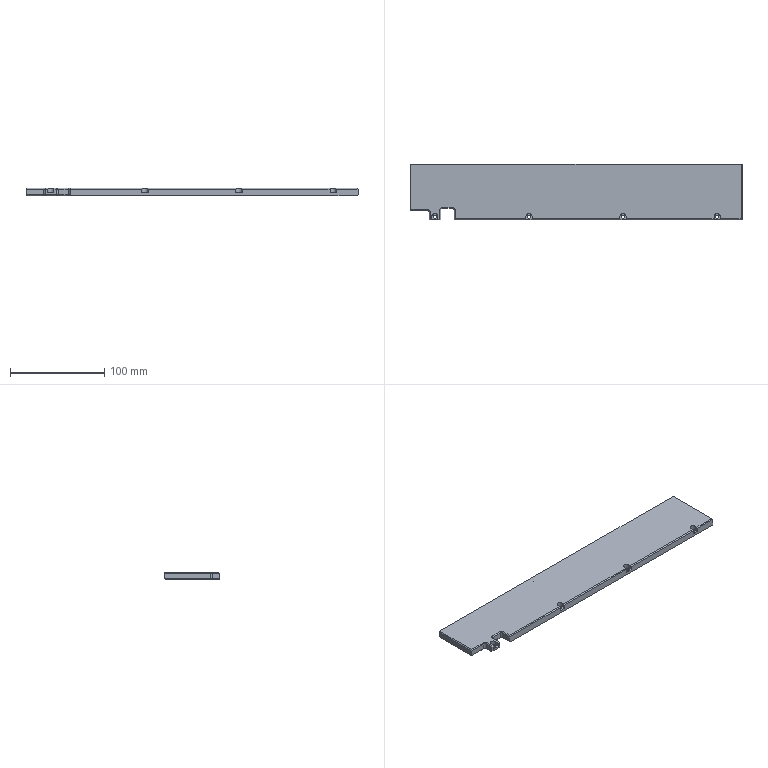CAM job | Mastercam | mm | 9 operations | part box 353 x 59 x 8
1. Contour (2D) | 7 - 4 平底刀
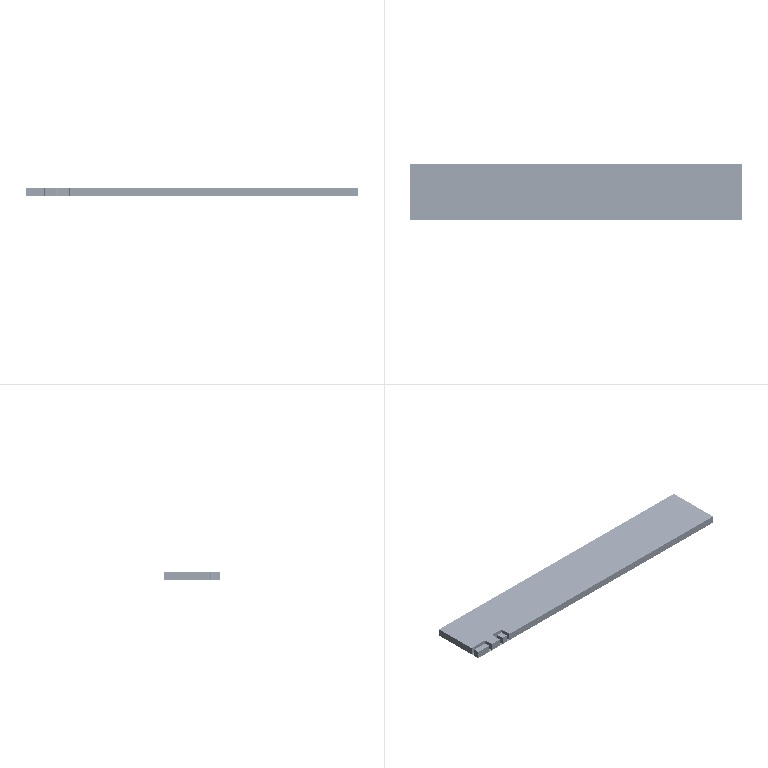2. Contour (Ramp) | 7 - 4 平底刀
3. Contour (2D) | 7 - 4 平底刀
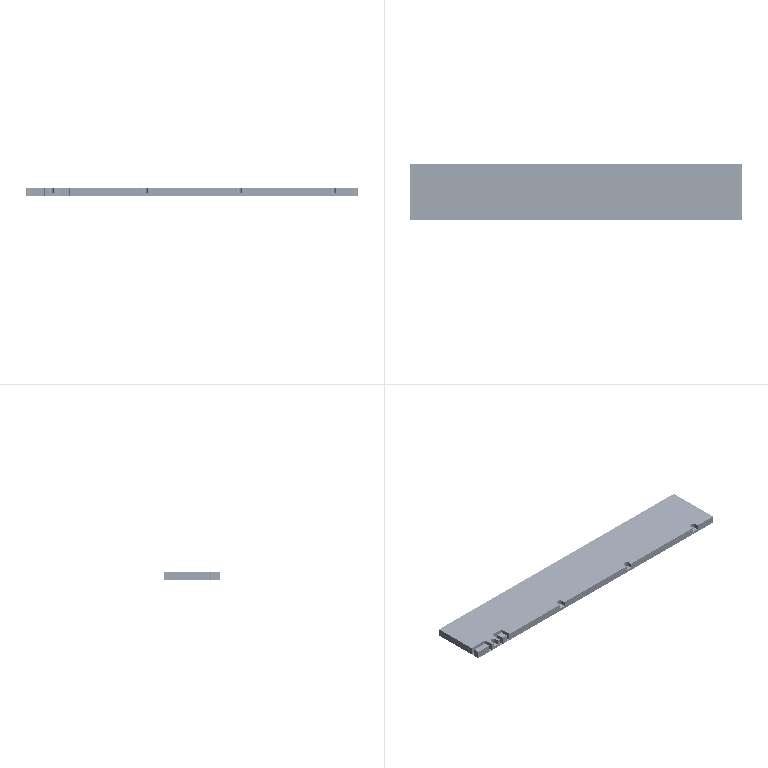4. Contour (2D chamfer) | 2 - 4定位倒角
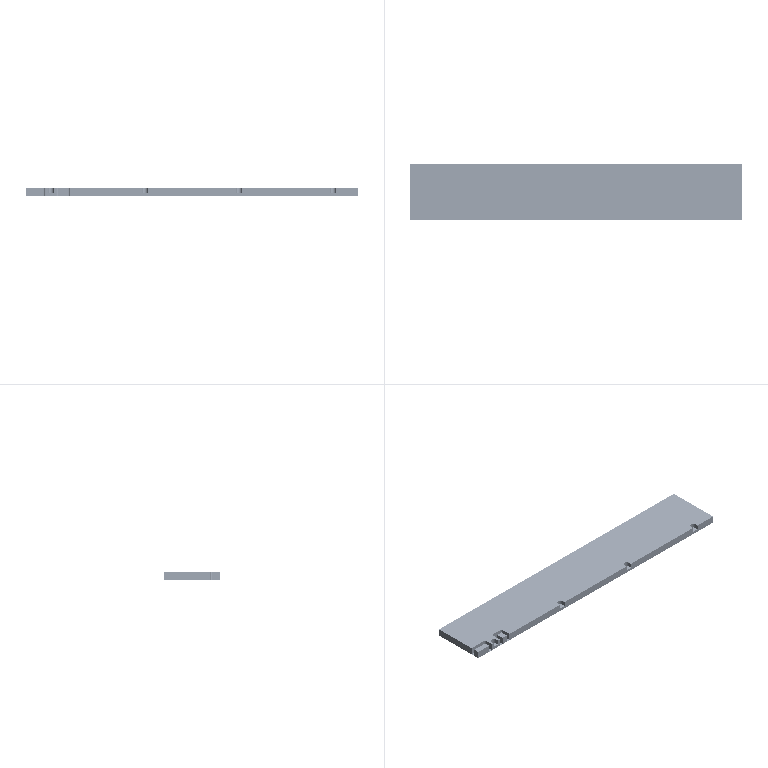5. Contour (2D chamfer) | 2 - 4定位倒角
6. Contour (2D) | 7 - 4 平底刀
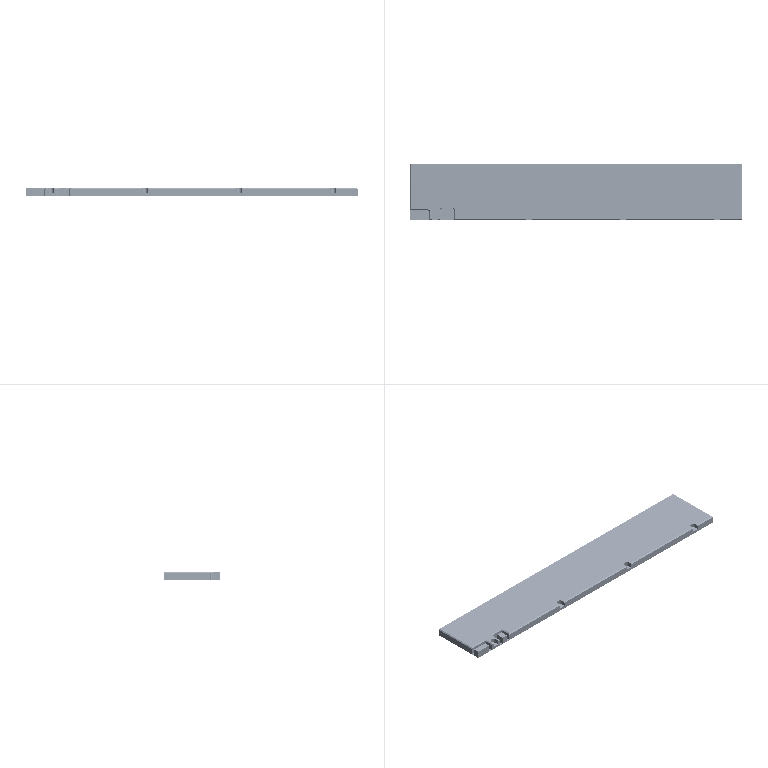7. Contour (2D chamfer) | 2 - 4定位倒角
8. Drill/Counterbore | 2 - 6定位倒角
9. Peck Drill | 12 - 2.5 钻头